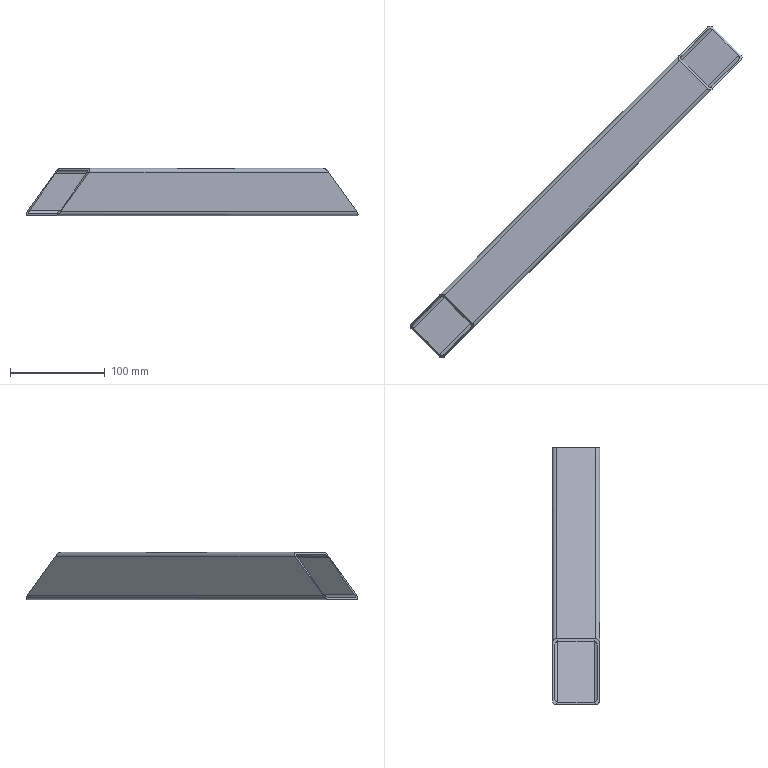Component | NX | SLID_FRAME_BEAM4_3 | 1 solid | 18 faces | volume 153600 mm3 | plane 10 | cylinder 8 | commonest cylinder face diameters 8 x8